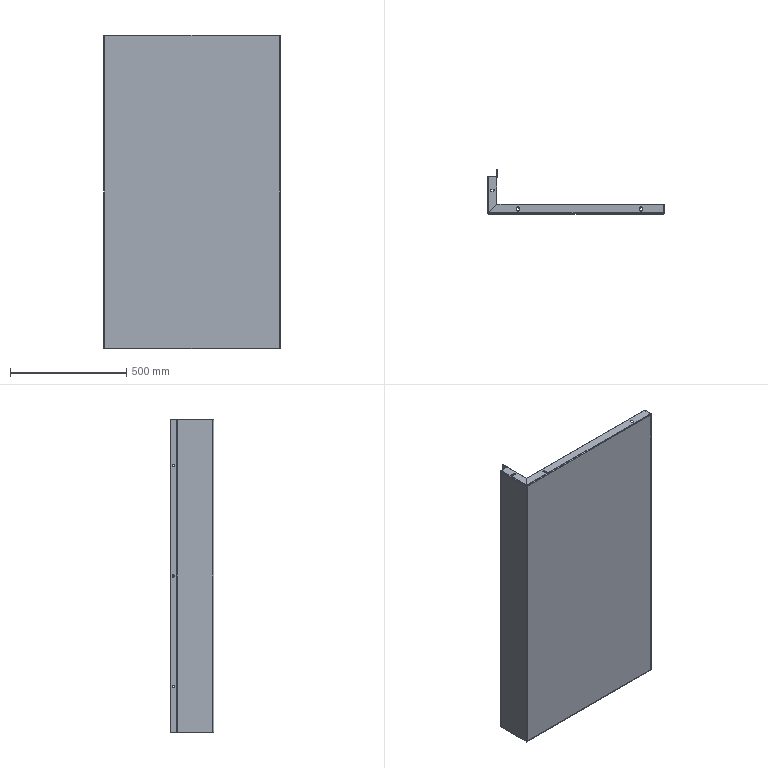Component | SolidWorks | FrontSidePlateAssembly-1_FrontSidePanel-1 | 1 solid | 147 faces | volume 2874121 mm3 | plane 80 | cylinder 59 | spline 8 | commonest cylinder face diameters 10 x37 4 x8 8 x8 9 x6 | material Plain Carbon Steel